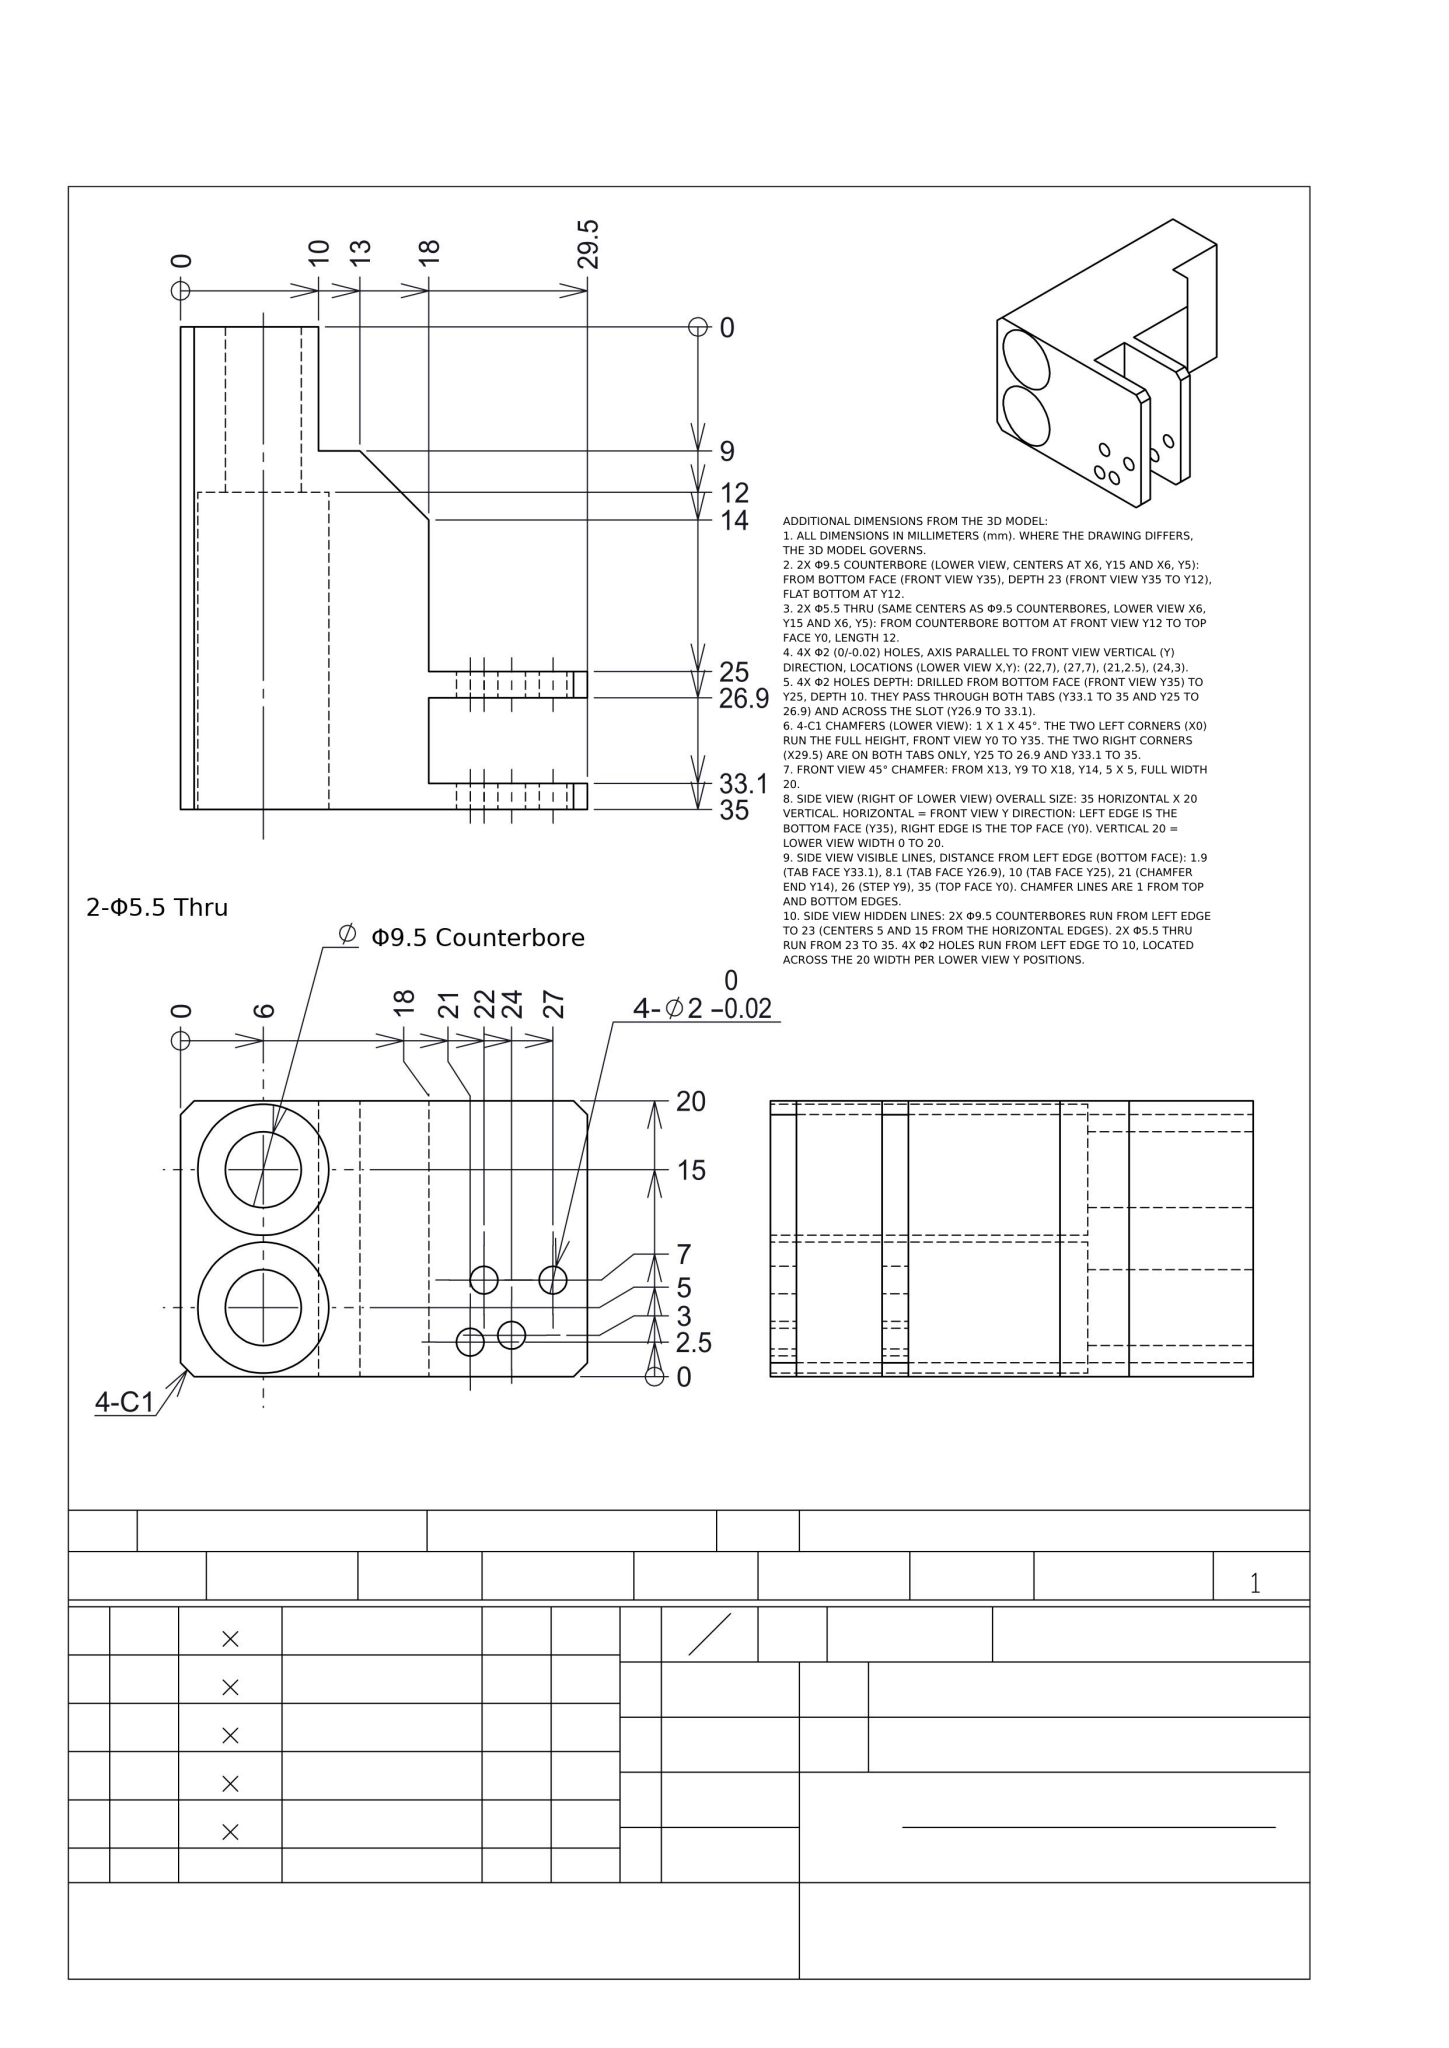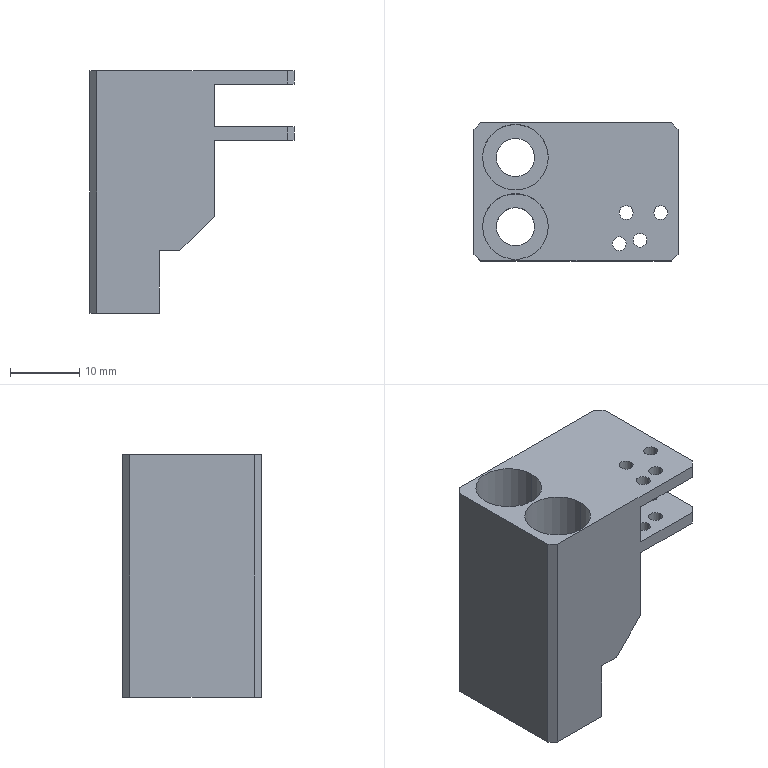Part | NX | mm | 1 solid | 47 faces | box 29.5 x 20 x 35 mm | volume 7867 mm3 | cylinder 24 | plane 23 | commonest cylinder face diameters 2 x16 9.5 x4 5.5 x4